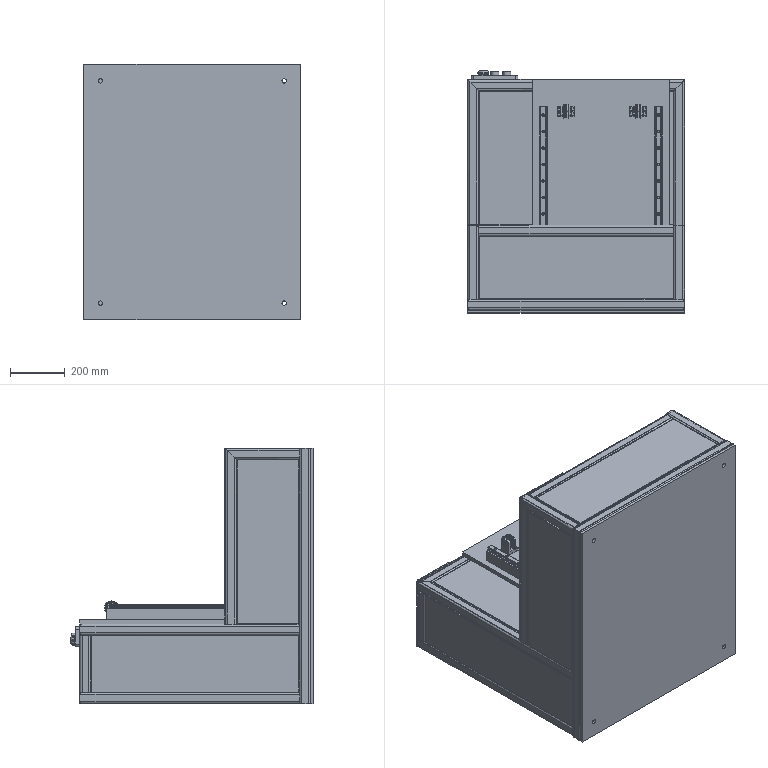Assembly | SolidWorks | mm | 31 component files | 55 solids | 3858 faces | box 791.5 x 883.5 x 930 mm | volume 28383413 mm3 | plane 2206 | cylinder 1246 | spline 340 | cone 46 | torus 20 | commonest cylinder face diameters 1 x194 3 x138 1.1 x120 16 x84 8 x76 1.6 x64 46.79 x62 6 x56
Bill of materials:
01000000A08005APulleyFixingSeat1(Battery)122 | 2 |  | Bracket with a rectangular base plate and two parallel upright lugs. Each lug has a large circular through-hole and chamfered top corners.
01000000A08017AAdjustingBeltPressureBlock(Battery)122 | 2 |  | Rectangular block whose top face has evenly spaced parallel ribs with rounded crests. Six elongated slots pass through the block.
01000000A08029AS5MPulley2(Battery)122 | 2 |  | Cylindrical toothed wheel with flanges on both ends and a small central through-bore.
ref7 | 1 |  | Thin, flat rectangular plate with no visible features.
ref26 | 2 |  | Thin, flat rectangular strip, shown standing on its long edge.
EmergencyStopSwitch122 | 1 |  | Rectangular block with a stepped (L-shaped) notch on one side. A cylindrical stem ends in a rounded, domed knob head.
F609ZZ(Battery)122 | 4 |  | Cylindrical ring with a thin flange at one end and a central through-bore.
ref7 | 1 | 1023 Carbon Steel Plate (SS) | Flat rectangular plate with sharp edges and no visible features.
ref26 | 1 |  | Thin, elongated, flat rectangular plate with no visible features.
GuideRailSliderEGH20CA122 | 4 | 6061 Alloy | Rectangular block with an open channel along its underside. The block has end caps, four holes on the top face, and small round bosses and a central hole on the end face.
ref10 | 2 |  | Long straight bar with a rectangular cross-section and four evenly spaced holes along its top face.
ref26 | 2 |  | Thin, flat rectangular panel, shown standing upright, with no visible features.
ref9 | 3 |  | Open right-triangle frame made from a bar of constant rectangular cross-section: a long vertical leg, a short horizontal base, and a long diagonal member joining them, leaving a triangular opening in the middle. Shaped like a gusset or bracket.
ref90 | 1 |  | Box-like open frame built from square or rectangular section members. The side profile is L-shaped: a tall rear section and a lower, deeper extended section. One large flat panel covers one side face. The frame has intermediate horizontal cross members, and small cylindrical protrusions sit on top and on one end.
ref7 | 1 | 1023 Carbon Steel Plate (SS) | Thin flat rectangular plate with straight edges and square corners.
Z-AxisLinearGuideEGH20CA-2-RL=550122 | 2 | 6061 Alloy | Long straight rail with a constant profiled cross-section. The sides have rounded grooves and recesses, and the base has chamfered corners and a shallow relief. A single row of evenly spaced holes, which appear counterbored, runs along the top face. Its shape resembles a profiled linear guide rail.
Mates:
1. coincident | Z-AxisLinearGuideEGH20CA-2-RL=550122-1 face at (-284.779, 464.741, 859.647) dir (0, 1, 0) | Z-AxisLinearGuideEGH20CA-2-RL=550122-2 face at (135.221, 464.741, 859.647) dir (0, 1, 0)
2. distance | Z-AxisLinearGuideEGH20CA-2-RL=550122-1 face at (-304.479, -135.259, 850.379) dir (-1, 0, 0) | FrameSupportPlate1122-1 face at (-334.479, -275.259, 805) dir (-1, 0, 0)
3. distance | Z-AxisLinearGuideEGH20CA-2-RL=550122-2 face at (115.521, -135.259, 850.379) dir (-1, 0, 0) | Z-AxisLinearGuideEGH20CA-2-RL=550122-1 face at (-284.479, -135.259, 847) dir (1, 0, 0)
4. distance | Z-AxisLinearGuideEGH20CA-2-RL=550122-1 face at (-284.779, 464.741, 859.647) dir (0, 1, 0) | FrameSupportPlate1122-1 face at (-334.479, 564.741, 805) dir (0, 1, 0)
5. coincident | GuideRailSliderEGH20CA122-2 face at (135.521, 25.152, 858.012) dir (-1, 0, 0) | Z-AxisLinearGuideEGH20CA-2-RL=550122-2 face at (135.521, -135.259, 857.953) dir (1, 0, 0)
6. coincident | Z-AxisLinearGuideEGH20CA-2-RL=550122-1 face at (-303.479, -135.259, 846) dir (0, 0, -1) | Z-AxisLinearGuideEGH20CA-2-RL=550122-2 face at (116.521, -135.259, 846) dir (0, 0, -1)
7. coincident | FrameSupportPlate1122-1 face at (-84.479, 144.741, 805) dir (0, 0, 1) | GuideRailSpacer122-1 face at (-294.479, 164.741, 805) dir (0, 0, -1)
8. coincident | Z-AxisLinearGuideEGH20CA-2-RL=550122-1 face at (-284.779, 464.741, 859.647) dir (0, 1, 0) | GuideRailSpacer122-1 face at (-309.479, 464.741, 846) dir (0, 1, 0)
9. width | GuideRailSpacer122-1 face at (-309.479, -135.259, 846) dir (-1, 0, 0) | GuideRailSpacer122-1 face at (-279.479, -135.259, 846) dir (1, 0, 0) | Z-AxisLinearGuideEGH20CA-2-RL=550122-1 face at (-284.479, -135.259, 847) dir (1, 0, 0) | Z-AxisLinearGuideEGH20CA-2-RL=550122-1 face at (-304.479, -135.259, 850.379) dir (-1, 0, 0)
10. coincident | Z-AxisLinearGuideEGH20CA-2-RL=550122-1 face at (-291.479, -135.259, 846) dir (0, 0, -1) | GuideRailSpacer122-1 face at (-294.479, 164.741, 846) dir (0, 0, 1)
11. coincident | FrameSupportPlate1122-1 face at (-84.479, 144.741, 805) dir (0, 0, 1) | GuideRailSpacer122-2 face at (125.521, 164.741, 805) dir (0, 0, -1)
12. coincident | GuideRailSpacer122-1 face at (-309.479, 464.741, 846) dir (0, 1, 0) | GuideRailSpacer122-2 face at (110.521, 464.741, 846) dir (0, 1, 0)
13. width | GuideRailSpacer122-2 face at (110.521, -135.259, 846) dir (-1, 0, 0) | GuideRailSpacer122-2 face at (140.521, -135.259, 846) dir (1, 0, 0) | Z-AxisLinearGuideEGH20CA-2-RL=550122-2 face at (135.521, -135.259, 847) dir (1, 0, 0) | Z-AxisLinearGuideEGH20CA-2-RL=550122-2 face at (115.521, -135.259, 850.379) dir (-1, 0, 0)
14. coincident | SlidingSupport1122-1 face at (-84.479, -49.348, 889.07) dir (0, 0, 1) | LiftingArm122-1 face at (-249.479, -124.348, 889.07) dir (0, 0, -1)
15. coincident | SlidingSupport1122-1 face at (-324.479, 25.652, 889.07) dir (0, 1, 0) | LiftingArm122-1 face at (-249.479, 25.652, 889.07) dir (0, 1, 0)
16. coincident | SlidingSupport1122-1 face at (-84.479, -49.348, 889.07) dir (0, 0, 1) | LiftingArm122-2 face at (-99.479, -124.348, 889.07) dir (0, 0, -1)
17. coincident | LiftingArm122-1 face at (-249.479, 25.652, 889.07) dir (0, 1, 0) | LiftingArm122-2 face at (-99.479, 25.652, 889.07) dir (0, 1, 0)
18. distance | LiftingArm122-2 face at (-99.479, 25.652, 889.07) dir (-1, 0, 0) | LiftingArm122-1 face at (-249.479, 25.652, 889.07) dir (-1, 0, 0)
19. coincident | SlidingSupport1122-1 face at (-84.479, -49.348, 889.07) dir (0, 0, 1) | LiftingArm122-3 face at (50.521, -124.348, 889.07) dir (0, 0, -1)
20. distance | LiftingArm122-3 face at (50.521, 25.652, 889.07) dir (-1, 0, 0) | LiftingArm122-2 face at (-99.479, 25.652, 889.07) dir (-1, 0, 0)
21. coincident | LiftingArm122-2 face at (-99.479, 25.652, 889.07) dir (0, 1, 0) | LiftingArm122-3 face at (50.521, 25.652, 889.07) dir (0, 1, 0)
22. distance | LiftingArm122-1 face at (-249.479, 25.652, 889.07) dir (-1, 0, 0) | SlidingSupport1122-1 face at (-324.479, -124.348, 889.07) dir (-1, 0, 0)
23. coincident | Z-AxisLinearGuideEGH20CA-2-RL=550122-2 face at (133.855, -135.259, 861.5) dir (0, 0, 1) | GuideRailSliderEGH20CA122-2 face at (133.896, 25.152, 861.5) dir (0, 0, -1)
24. coincident | Z-AxisLinearGuideEGH20CA-2-RL=550122-1 face at (-284.479, -135.259, 857.953) dir (1, 0, 0) | GuideRailSliderEGH20CA122-3 face at (-284.479, 25.152, 858.012) dir (-1, 0, 0)
25. coincident | Z-AxisLinearGuideEGH20CA-2-RL=550122-1 face at (-286.145, -135.259, 861.5) dir (0, 0, 1) | GuideRailSliderEGH20CA122-3 face at (-286.104, 25.152, 861.5) dir (0, 0, -1)
26. coincident | GuideRailSliderEGH20CA122-2 face at (106.891, 25.652, 873.07) dir (0, 1, 0) | GuideRailSliderEGH20CA122-3 face at (-313.109, 25.652, 873.07) dir (0, 1, 0)
27. coincident | GuideRailSliderEGH20CA122-1 face at (-301.409, -63.948, 874.07) dir (0, 0, 1) | GuideRailSliderEGH20CA122-3 face at (-301.409, 15.152, 874.07) dir (0, 0, 1)
28. coincident | GuideRailSliderEGH20CA122-1 face at (-315.409, -63.948, 873.07) dir (-1, 0, 0) | GuideRailSliderEGH20CA122-3 face at (-315.409, 15.152, 873.07) dir (-1, 0, 0)
29. distance | GuideRailSliderEGH20CA122-1 face at (-313.109, -53.448, 873.07) dir (0, 1, 0) | GuideRailSliderEGH20CA122-3 face at (-313.109, -43.448, 873.07) dir (0, -1, 0)
30. coincident | GuideRailSliderEGH20CA122-1 face at (-313.109, -122.548, 873.07) dir (0, -1, 0) | GuideRailSliderEGH20CA122-5 face at (106.891, -122.548, 873.07) dir (0, -1, 0)
31. coincident | GuideRailSliderEGH20CA122-2 face at (104.591, 15.152, 873.07) dir (-1, 0, 0) | GuideRailSliderEGH20CA122-5 face at (104.591, -63.948, 873.07) dir (-1, 0, 0)
32. coincident | GuideRailSliderEGH20CA122-2 face at (118.591, 15.152, 874.07) dir (0, 0, 1) | GuideRailSliderEGH20CA122-5 face at (118.591, -63.948, 874.07) dir (0, 0, 1)
33. coincident | GuideRailSliderEGH20CA122-5 face at (118.591, -63.948, 874.07) dir (0, 0, 1) | SlidingSupport1122-1 face at (-84.479, -49.348, 874.07) dir (0, 0, -1)
34. width | FrameSupportPlate1122-1 face at (-334.479, -275.259, 805) dir (-1, 0, 0) | FrameSupportPlate1122-1 face at (165.521, -275.259, 805) dir (1, 0, 0) | SlidingSupport1122-1 face at (155.521, -124.348, 889.07) dir (1, 0, 0) | SlidingSupport1122-1 face at (-324.479, -124.348, 889.07) dir (-1, 0, 0)
35. coincident | GuideRailSliderEGH20CA122-3 face at (-313.109, 25.652, 873.07) dir (0, 1, 0) | SlidingSupport1122-1 face at (-324.479, 25.652, 889.07) dir (0, 1, 0)
36. coincident | FrameSupportPlate1122-1 face at (-84.479, 144.741, 805) dir (0, 0, 1) | 01000000A08005APulleyFixingSeat1(Battery)122-1 face at (-230.479, 467.741, 805) dir (0, 0, -1)
37. coincident | FrameSupportPlate1122-1 face at (-84.479, 144.741, 805) dir (0, 0, 1) | 01000000A08005APulleyFixingSeat1(Battery)122-2 face at (32.521, 467.741, 805) dir (0, 0, -1)
38. concentric | 01000000A08005APulleyFixingSeat1(Battery)122-1 face at (-230.479, 448.741, 848.5) dir (1, 0, 0) r 12 | 01000000A08029AS5MPulley2(Battery)122-1 face at (-212.479, 448.741, 848.5) dir (-1, 0, 0) r 4.5
39. width | 01000000A08005APulleyFixingSeat1(Battery)122-1 face at (-230.479, 429.741, 865) dir (-1, 0, 0) | 01000000A08005APulleyFixingSeat1(Battery)122-1 face at (-194.479, 429.741, 865) dir (1, 0, 0) | 01000000A08029AS5MPulley2(Battery)122-1 face at (-202.479, 474.241, 848.5) dir (1, 0, 0) | 01000000A08029AS5MPulley2(Battery)122-1 face at (-222.479, 453.241, 848.5) dir (-1, 0, 0)
40. concentric | 01000000A08005APulleyFixingSeat1(Battery)122-2 face at (32.521, 448.741, 848.5) dir (1, 0, 0) r 12 | 01000000A08029AS5MPulley2(Battery)122-2 face at (50.521, 448.741, 848.5) dir (-1, 0, 0) r 4.5
41. width | 01000000A08029AS5MPulley2(Battery)122-2 face at (40.521, 453.241, 848.5) dir (-1, 0, 0) | 01000000A08029AS5MPulley2(Battery)122-2 face at (60.521, 474.241, 848.5) dir (1, 0, 0) | 01000000A08005APulleyFixingSeat1(Battery)122-2 face at (68.521, 429.741, 865) dir (1, 0, 0) | 01000000A08005APulleyFixingSeat1(Battery)122-2 face at (32.521, 429.741, 865) dir (-1, 0, 0)
42. coincident | 01000000A08005APulleyFixingSeat1(Battery)122-1 face at (-230.479, 429.741, 865) dir (-1, 0, 0) | F609ZZ(Battery)122-1 face at (-230.479, 438.613, 854.936) dir (1, 0, 0)
43. concentric | 01000000A08005APulleyFixingSeat1(Battery)122-1 face at (-230.479, 448.741, 848.5) dir (1, 0, 0) r 12 | F609ZZ(Battery)122-1 face at (-231.979, 448.741, 848.5) dir (-1, 0, 0) r 12
44. coincident | 01000000A08005APulleyFixingSeat1(Battery)122-1 face at (-194.479, 429.741, 865) dir (1, 0, 0) | F609ZZ(Battery)122-2 face at (-194.479, 438.925, 855.403) dir (-1, 0, 0)
45. concentric | 01000000A08005APulleyFixingSeat1(Battery)122-1 face at (-230.479, 448.741, 848.5) dir (1, 0, 0) r 12 | F609ZZ(Battery)122-2 face at (-192.979, 448.741, 848.5) dir (1, 0, 0) r 12
46. coincident | 01000000A08005APulleyFixingSeat1(Battery)122-2 face at (32.521, 429.741, 865) dir (-1, 0, 0) | F609ZZ(Battery)122-3 face at (32.521, 438.613, 854.936) dir (1, 0, 0)
47. concentric | 01000000A08005APulleyFixingSeat1(Battery)122-2 face at (32.521, 448.741, 848.5) dir (1, 0, 0) r 12 | F609ZZ(Battery)122-3 face at (31.021, 448.741, 848.5) dir (-1, 0, 0) r 12
48. coincident | 01000000A08005APulleyFixingSeat1(Battery)122-2 face at (68.521, 429.741, 865) dir (1, 0, 0) | F609ZZ(Battery)122-4 face at (68.521, 438.925, 855.403) dir (-1, 0, 0)
49. concentric | 01000000A08005APulleyFixingSeat1(Battery)122-2 face at (32.521, 448.741, 848.5) dir (1, 0, 0) r 12 | F609ZZ(Battery)122-4 face at (70.021, 448.741, 848.5) dir (1, 0, 0) r 12
50. coincident | SlidingSupport1122-1 face at (-84.479, -49.348, 874.07) dir (0, 0, -1) | 01000000A08017AAdjustingBeltPressureBlock(Battery)122-1 face at (-227.479, -26.348, 874.07) dir (0, 0, 1)
51. distance | 01000000A08017AAdjustingBeltPressureBlock(Battery)122-1 face at (-227.479, -49.348, 866.07) dir (0, -1, 0) | SlidingSupport1122-1 face at (-324.479, -124.348, 889.07) dir (0, -1, 0)
52. coincident | SlidingSupport1122-1 face at (-84.479, -49.348, 874.07) dir (0, 0, -1) | 01000000A08017AAdjustingBeltPressureBlock(Battery)122-2 face at (35.521, -21.348, 874.07) dir (0, 0, 1)
53. coincident | 01000000A08017AAdjustingBeltPressureBlock(Battery)122-1 face at (-227.479, -4.348, 874.07) dir (0, 1, 0) | 01000000A08017AAdjustingBeltPressureBlock(Battery)122-2 face at (35.521, -4.348, 874.07) dir (0, 1, 0)
54. coincident | FrameSupportPlate1122-1 face at (-84.479, 144.741, 790) dir (0, 0, -1) | LoadingRack122-1 face at (-561.479, 543.241, 790) dir (0, 0, 1)
55. parallel | FrameSupportPlate1122-1 face at (-334.479, -275.259, 805) dir (0, -1, 0) | LoadingRack122-1 face at (212.521, -276.759, 1410) dir (0, -1, 0)
56. coincident | FrameSupportPlate1122-1 face at (-334.479, 564.741, 805) dir (0, 1, 0) | LoadingRack122-1 face at (-549.479, 564.741, 1410) dir (0, 1, 0)
57. distance | FrameSupportPlate1122-1 face at (165.521, -275.259, 805) dir (1, 0, 0) | LoadingRack122-1 face at (180.521, -256.759, 758) dir (-1, 0, 0)
58. coincident | LoadingRack122-1 face at (-569.479, 543.241, 782) dir (-1, 0, 0) | ElectricalBoxSideDoor122-1 face at (-569.479, 143.241, 645) dir (-1, 0, 0)
59. coincident | LoadingRack122-1 face at (-561.479, 523.241, 770) dir (0, -1, 0) | ElectricalBoxSideDoor122-1 face at (-567.979, 523.241, 645) dir (0, 1, 0)
60. coincident | LoadingRack122-1 face at (-561.479, 543.241, 540) dir (0, 0, 1) | ElectricalBoxSideDoor122-1 face at (-567.979, 143.241, 540) dir (0, 0, -1)
61. coincident | LoadingRack122-1 face at (220.521, 555.241, 770) dir (1, 0, 0) | ElectricalBoxSideDoor122-2 face at (220.521, 143.241, 645) dir (1, 0, 0)
62. coincident | LoadingRack122-1 face at (188.521, -256.759, 750) dir (0, 0, -1) | ElectricalBoxSideDoor122-2 face at (219.021, 143.241, 750) dir (0, 0, 1)
63. coincident | LoadingRack122-1 face at (188.521, -236.759, 1410) dir (0, 1, 0) | ElectricalBoxSideDoor122-2 face at (219.021, -236.759, 645) dir (0, -1, 0)
64. coincident | LoadingRack122-1 face at (-569.479, 25.241, 770) dir (-1, 0, 0) | LeftAndRightSidePlates122-1 face at (-569.479, -121.759, 1090) dir (1, 0, 0)
65. coincident | LoadingRack122-1 face at (-537.479, 13.241, 1390) dir (0, 0, -1) | LeftAndRightSidePlates122-1 face at (-569.479, -121.759, 1390) dir (0, 0, 1)
66. coincident | LoadingRack122-1 face at (-537.479, -236.759, 520) dir (0, 1, 0) | LeftAndRightSidePlates122-1 face at (-569.479, -236.759, 1090) dir (0, -1, 0)
67. coincident | LoadingRack122-1 face at (220.521, -256.759, 782) dir (1, 0, 0) | LeftAndRightSidePlates122-2 face at (220.521, -121.759, 1090) dir (1, 0, 0)
68. coincident | LoadingRack122-1 face at (212.521, 13.241, 1390) dir (0, 0, -1) | LeftAndRightSidePlates122-2 face at (219.021, -121.759, 1390) dir (0, 0, 1)
69. coincident | LoadingRack122-1 face at (188.521, -236.759, 1410) dir (0, 1, 0) | LeftAndRightSidePlates122-2 face at (219.021, -236.759, 1090) dir (0, -1, 0)
70. coincident | LoadingRack122-1 face at (-549.479, 1.241, 1430) dir (0, 0, 1) | FrontDoorPlate122-1 face at (-174.479, -121.759, 1430) dir (0, 0, 1)
71. coincident | LoadingRack122-1 face at (-549.479, -6.759, 1422) dir (0, -1, 0) | FrontDoorPlate122-1 face at (-174.479, -6.759, 1428.5) dir (0, 1, 0)
72. coincident | LoadingRack122-1 face at (-529.479, 13.241, 1398) dir (1, 0, 0) | FrontDoorPlate122-1 face at (-529.479, -121.759, 1428.5) dir (-1, 0, 0)
73. coincident | LoadingRack122-1 face at (200.521, 555.241, 790) dir (0, 0, 1) | ElectricalBoxPlate2122-1 face at (-174.479, 278.241, 790) dir (0, 0, 1)
74. coincident | LoadingRack122-1 face at (200.521, 523.241, 758) dir (0, -1, 0) | ElectricalBoxPlate2122-1 face at (-174.479, 523.241, 788.5) dir (0, 1, 0)
75. coincident | LoadingRack122-1 face at (-529.479, 543.241, 758) dir (1, 0, 0) | ElectricalBoxPlate2122-1 face at (-529.479, 278.241, 788.5) dir (-1, 0, 0)
76. coincident | LoadingRack122-1 face at (-549.479, 564.741, 1410) dir (0, 1, 0) | EmergencyStopSwitch122-1 face at (-497.479, 564.741, 748) dir (0, 1, 0)
77. concentric | LoadingRack122-1 sketch segment at (-512.479, 564.741, 730) dir (0, 1, 0) r 10.32 | EmergencyStopSwitch122-1 face at (-512.479, 564.741, 730) dir (0, -1, 0) r 11